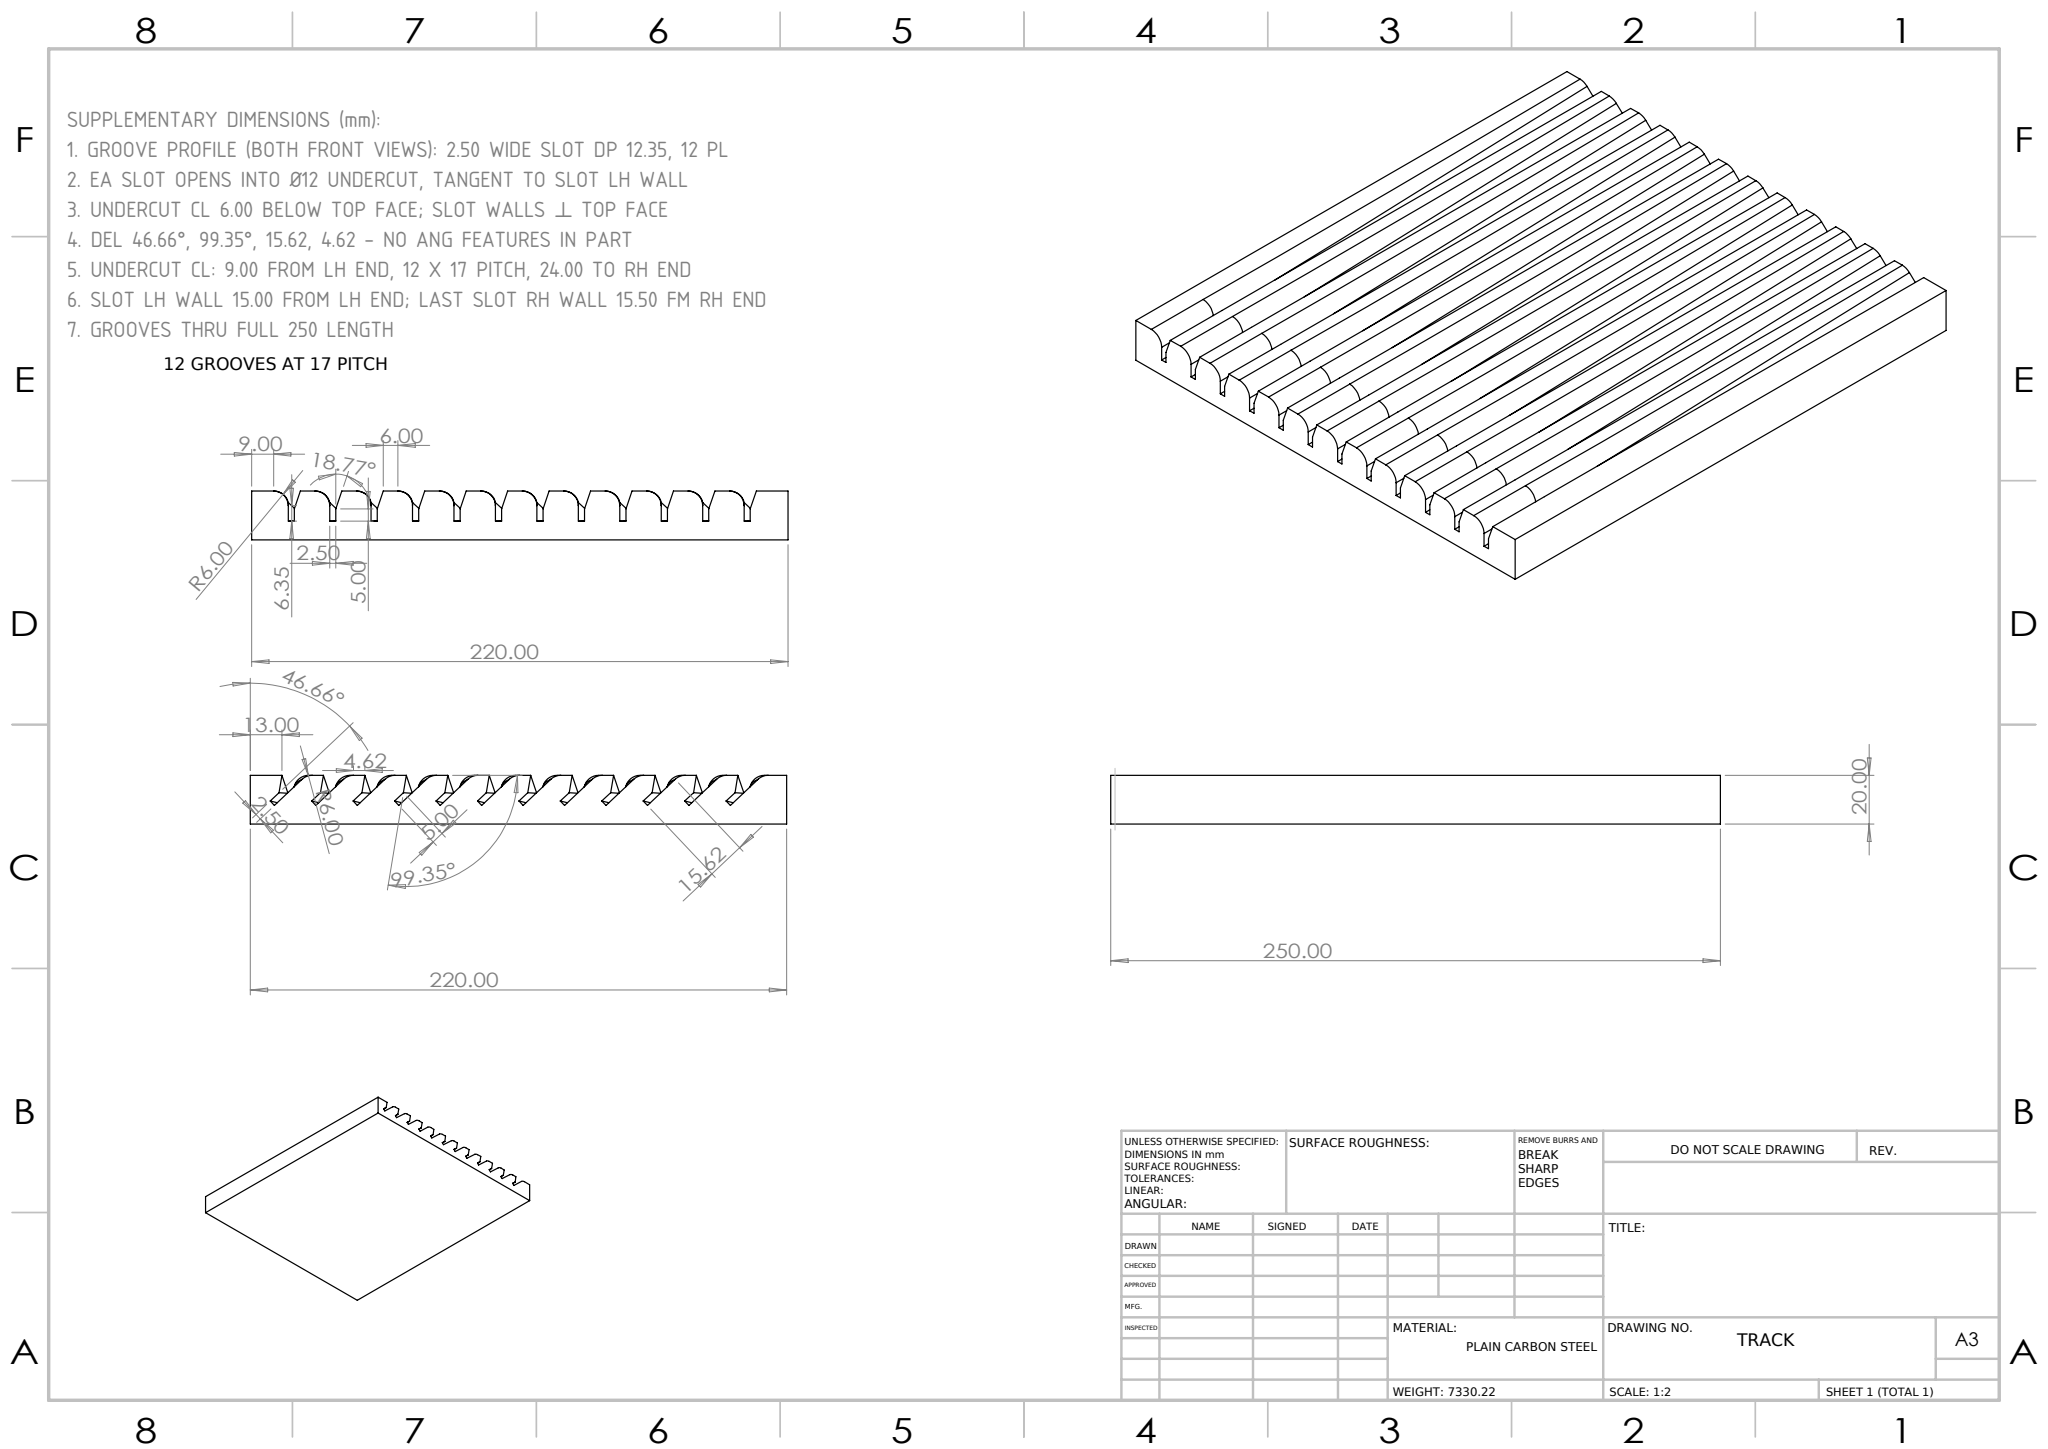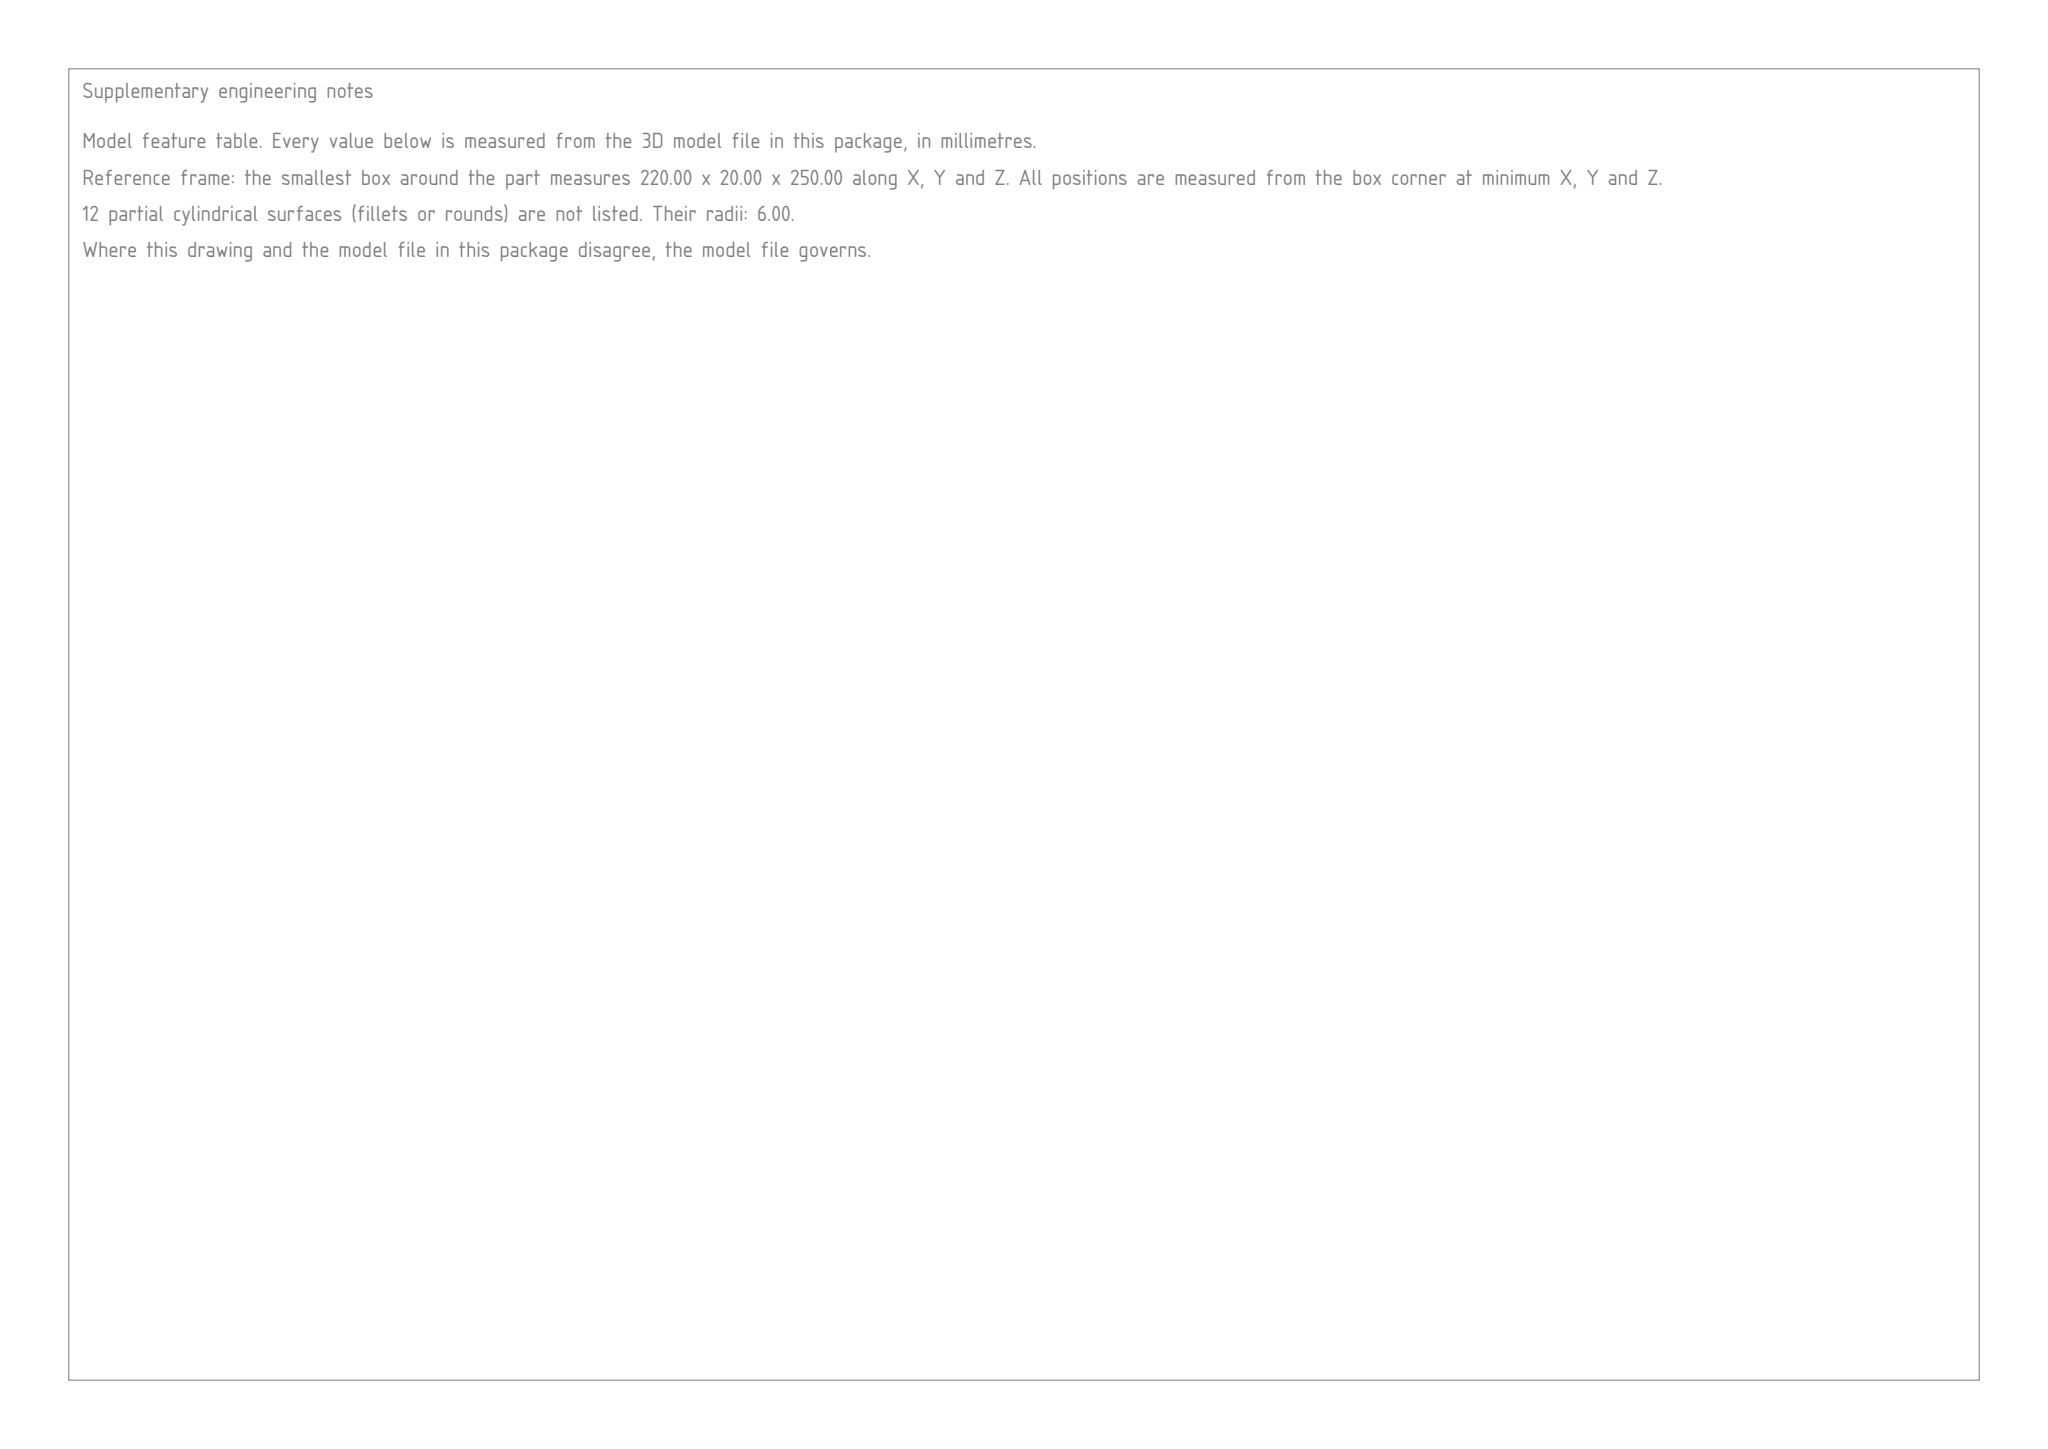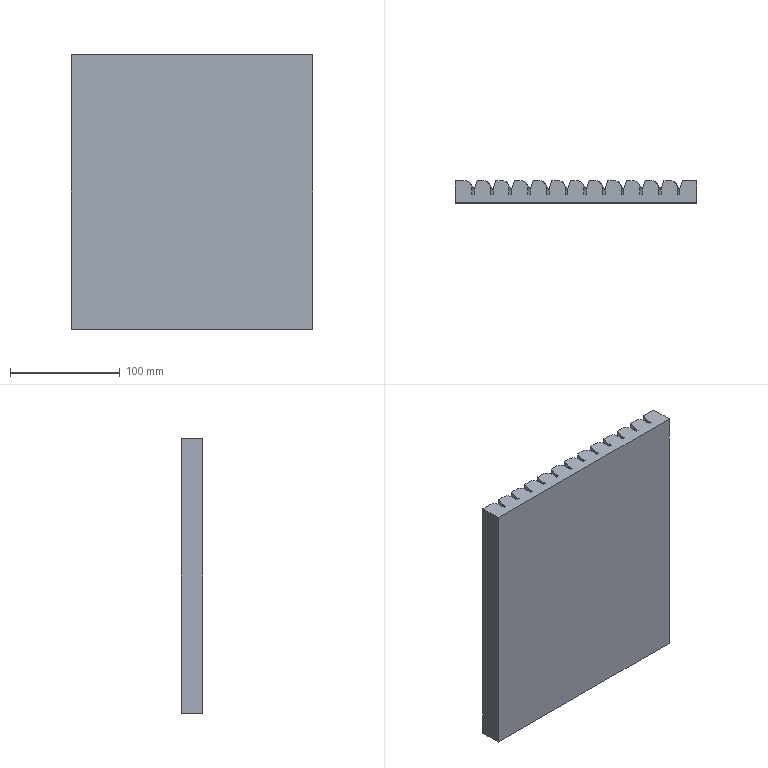Part | SolidWorks | mm | 1 solid | 138 faces | box 220 x 20 x 250 mm | volume 939773 mm3 | plane 66 | spline 60 | cylinder 12 | commonest cylinder face diameters 12 x12
build123d program:
from build123d import *

# Parameters (mm, degrees)
BOSS_EXTRUDE1_DEPTH = 30
FILLET1_R           = 6


with BuildPart() as part:
    # Sketch1 → Loft2 section 0
    with BuildSketch(Plane.XY):
        with BuildLine():
            Line((0, 0), (0, 20))
            Line((0, 20), (10, 20))
            Line((10, 20), (23.091, 7.646))
            Line((23.091, 7.646), (24.807, 9.464))
            Line((24.807, 9.464), (21.17, 12.896))
            Line((21.17, 12.896), (20, 20))
            Line((20, 20), (27, 20))
            Line((27, 20), (40.091, 7.646))
            Line((40.091, 7.646), (41.807, 9.464))
            Line((41.807, 9.464), (38.17, 12.896))
            Line((38.17, 12.896), (37, 20))
            Line((37, 20), (44, 20))
            Line((44, 20), (57.091, 7.646))
            Line((57.091, 7.646), (58.807, 9.464))
            Line((58.807, 9.464), (55.17, 12.896))
            Line((55.17, 12.896), (54, 20))
            Line((54, 20), (61, 20))
            Line((61, 20), (74.091, 7.646))
            Line((74.091, 7.646), (75.807, 9.464))
            Line((75.807, 9.464), (72.17, 12.896))
            Line((72.17, 12.896), (71, 20))
            Line((71, 20), (78, 20))
            Line((78, 20), (91.091, 7.646))
            Line((91.091, 7.646), (92.807, 9.464))
            Line((92.807, 9.464), (89.17, 12.896))
            Line((89.17, 12.896), (88, 20))
            Line((88, 20), (95, 20))
            Line((95, 20), (108.091, 7.646))
            Line((108.091, 7.646), (109.807, 9.464))
            Line((109.807, 9.464), (106.17, 12.896))
            Line((106.17, 12.896), (105, 20))
            Line((105, 20), (112, 20))
            Line((112, 20), (125.091, 7.646))
            Line((125.091, 7.646), (126.807, 9.464))
            Line((126.807, 9.464), (123.17, 12.896))
            Line((123.17, 12.896), (122, 20))
            Line((122, 20), (129, 20))
            Line((129, 20), (142.091, 7.646))
            Line((142.091, 7.646), (143.807, 9.464))
            Line((143.807, 9.464), (140.17, 12.896))
            Line((140.17, 12.896), (139, 20))
            Line((139, 20), (146, 20))
            Line((146, 20), (159.091, 7.646))
            Line((159.091, 7.646), (160.807, 9.464))
            Line((160.807, 9.464), (157.17, 12.896))
            Line((157.17, 12.896), (156, 20))
            Line((156, 20), (163, 20))
            Line((163, 20), (176.091, 7.646))
            Line((176.091, 7.646), (177.807, 9.464))
            Line((177.807, 9.464), (174.17, 12.896))
            Line((174.17, 12.896), (173, 20))
            Line((173, 20), (180, 20))
            Line((180, 20), (193.091, 7.646))
            Line((193.091, 7.646), (194.807, 9.464))
            Line((194.807, 9.464), (191.17, 12.896))
            Line((191.17, 12.896), (190, 20))
            Line((190, 20), (197, 20))
            Line((197, 20), (210.091, 7.646))
            Line((210.091, 7.646), (211.807, 9.464))
            Line((211.807, 9.464), (208.17, 12.896))
            Line((208.17, 12.896), (207, 20))
            Line((207, 20), (220, 20))
            Line((220, 20), (220, 0))
            Line((220, 0), (0, 0))
        make_face()
    # Sketch2 → Loft2 section 1
    with BuildSketch(Plane.XY.offset(220)):
        with BuildLine():
            Line((0, 0), (0, 20))
            Line((0, 20), (15, 20))
            Line((15, 20), (15, 7.646))
            Line((15, 7.646), (17.5, 7.646))
            Line((17.5, 7.646), (17.5, 12.646))
            Line((17.5, 12.646), (20, 20))
            Line((20, 20), (32, 20))
            Line((32, 20), (32, 7.646))
            Line((32, 7.646), (34.5, 7.646))
            Line((34.5, 7.646), (34.5, 12.646))
            Line((34.5, 12.646), (37, 20))
            Line((37, 20), (49, 20))
            Line((49, 20), (49, 7.646))
            Line((49, 7.646), (51.5, 7.646))
            Line((51.5, 7.646), (51.5, 12.646))
            Line((51.5, 12.646), (54, 20))
            Line((54, 20), (66, 20))
            Line((66, 20), (66, 7.646))
            Line((66, 7.646), (68.5, 7.646))
            Line((68.5, 7.646), (68.5, 12.646))
            Line((68.5, 12.646), (71, 20))
            Line((71, 20), (83, 20))
            Line((83, 20), (83, 7.646))
            Line((83, 7.646), (85.5, 7.646))
            Line((85.5, 7.646), (85.5, 12.646))
            Line((85.5, 12.646), (88, 20))
            Line((88, 20), (100, 20))
            Line((100, 20), (100, 7.646))
            Line((100, 7.646), (102.5, 7.646))
            Line((102.5, 7.646), (102.5, 12.646))
            Line((102.5, 12.646), (105, 20))
            Line((105, 20), (117, 20))
            Line((117, 20), (117, 7.646))
            Line((117, 7.646), (119.5, 7.646))
            Line((119.5, 7.646), (119.5, 12.646))
            Line((119.5, 12.646), (122, 20))
            Line((122, 20), (134, 20))
            Line((134, 20), (134, 7.646))
            Line((134, 7.646), (136.5, 7.646))
            Line((136.5, 7.646), (136.5, 12.646))
            Line((136.5, 12.646), (139, 20))
            Line((139, 20), (151, 20))
            Line((151, 20), (151, 7.646))
            Line((151, 7.646), (153.5, 7.646))
            Line((153.5, 7.646), (153.5, 12.646))
            Line((153.5, 12.646), (156, 20))
            Line((156, 20), (168, 20))
            Line((168, 20), (168, 7.646))
            Line((168, 7.646), (170.5, 7.646))
            Line((170.5, 7.646), (170.5, 12.646))
            Line((170.5, 12.646), (173, 20))
            Line((173, 20), (185, 20))
            Line((185, 20), (185, 7.646))
            Line((185, 7.646), (187.5, 7.646))
            Line((187.5, 7.646), (187.5, 12.646))
            Line((187.5, 12.646), (190, 20))
            Line((190, 20), (202, 20))
            Line((202, 20), (202, 7.646))
            Line((202, 7.646), (204.5, 7.646))
            Line((204.5, 7.646), (204.5, 12.646))
            Line((204.5, 12.646), (207, 20))
            Line((207, 20), (220, 20))
            Line((220, 20), (220, 0))
            Line((220, 0), (0, 0))
        make_face()
    loft()

    # Sketch3 → Boss-Extrude1 (add)
    with BuildSketch(Plane.XY.offset(220)):
        Polygon((0, 0), (220, 0), (220, 20), (207, 20), (204.5, 12.646), (204.5, 7.646), (202, 7.646), (202, 20), (190, 20), (187.5, 12.646), (187.5, 7.646), (185, 7.646), (185, 20), (173, 20), (170.5, 12.646), (170.5, 7.646), (168, 7.646), (168, 20), (156, 20), (153.5, 12.646), (153.5, 7.646), (151, 7.646), (151, 20), (139, 20), (136.5, 12.646), (136.5, 7.646), (134, 7.646), (134, 20), (122, 20), (119.5, 12.646), (119.5, 7.646), (117, 7.646), (117, 20), (105, 20), (102.5, 12.646), (102.5, 7.646), (100, 7.646), (100, 20), (88, 20), (85.5, 12.646), (85.5, 7.646), (83, 7.646), (83, 20), (71, 20), (68.5, 12.646), (68.5, 7.646), (66, 7.646), (66, 20), (54, 20), (51.5, 12.646), (51.5, 7.646), (49, 7.646), (49, 20), (37, 20), (34.5, 12.646), (34.5, 7.646), (32, 7.646), (32, 20), (20, 20), (17.5, 12.646), (17.5, 7.646), (15, 7.646), (15, 20), (0, 20), align=None)
    extrude(amount=BOSS_EXTRUDE1_DEPTH)

    # Fillet1
    fillet1_edges = [part.edges().sort_by_distance(p)[0] for p in [
        (199.5, 20, 110),
        (182.5, 20, 110),
        (165.5, 20, 110),
        (148.5, 20, 110),
        (131.5, 20, 110),
        (114.5, 20, 110),
        (97.5, 20, 110),
        (80.5, 20, 110),
        (63.5, 20, 110),
        (46.5, 20, 110),
        (29.5, 20, 110),
        (12.5, 20, 110),
    ]]
    fillet(fillet1_edges, radius=FILLET1_R)


solid = part.part